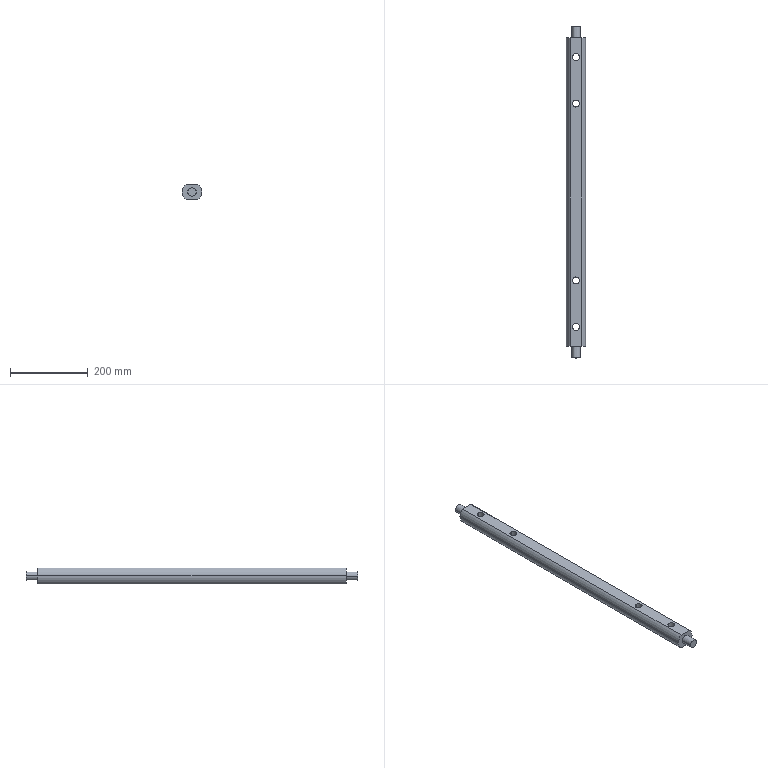Component | SolidWorks | FixedFrame-1 | 1 solid | 21 faces | box 50 x 856 x 40 mm | volume 1382352 mm3 | cylinder 15 | plane 6 | commonest cylinder face diameters 18 x8 22 x4 50 x3
build123d program:
from build123d import *

# Parameters (mm, degrees)
SKETCH1_R           = 25
BOSS_EXTRUDE1_DEPTH = 398
SKETCH2_R           = 11
BOSS_EXTRUDE2_DEPTH = 30
SKETCH3_W           = 60
SKETCH3_H           = 14.79
CUT_EXTRUDE1_DEPTH  = 827.756
SKETCH4_R           = 9
CUT_EXTRUDE2_DEPTH  = 656


with BuildPart() as part:
    # Sketch1 → Boss-Extrude1 (new, symmetric)
    with BuildSketch(Plane.XY):
        Circle(SKETCH1_R)
    extrude(amount=BOSS_EXTRUDE1_DEPTH, both=True)

    # Sketch2 → Boss-Extrude2 (add)
    with BuildSketch(Plane.XY.offset(398)):
        Circle(SKETCH2_R)
    extrude(amount=BOSS_EXTRUDE2_DEPTH)

    # Mirror1: part across plane


with BuildPart() as part_1:
    add(part.part)
    add(part.part.mirror(Plane.XY))

    # Sketch3 → Cut-Extrude1 (cut, through all)
    with BuildSketch(Plane.XY.offset(398)):
        with Locations((0, 27.395)):
            Rectangle(SKETCH3_W, SKETCH3_H)
        with Locations((0, -27.395)):
            Rectangle(SKETCH3_W, SKETCH3_H)
    extrude(amount=-CUT_EXTRUDE1_DEPTH, mode=Mode.SUBTRACT)

    # Sketch4 → Cut-Extrude2 (cut)
    with BuildSketch(Plane(origin=(0, 20, 0), x_dir=(1, 0, 0), z_dir=(0, 1, 0))):
        with Locations(Location((0, -228, 0), (0, 0, 270))):
            Circle(SKETCH4_R)
        with Locations(Location((0, -348, 0), (0, 0, 270))):
            Circle(SKETCH4_R)
        with Locations(Location((0, 348, 0), (0, 0, 270))):
            Circle(SKETCH4_R)
        with Locations(Location((0, 228, 0), (0, 0, 270))):
            Circle(SKETCH4_R)
    extrude(amount=-CUT_EXTRUDE2_DEPTH, mode=Mode.SUBTRACT)


solid = part_1.part

# Placed as in the assembly
solid = solid.moved(Location((-917, 0, -160), (90, 0, 0)))
STEP:
#1=COLOUR_RGB('',0.7922,0.8196,0.9333);
#2=FILL_AREA_STYLE_COLOUR('',#1);
#3=FILL_AREA_STYLE('',(#2));
#4=SURFACE_STYLE_FILL_AREA(#3);
#5=SURFACE_SIDE_STYLE('',(#4));
#6=SURFACE_STYLE_USAGE(.BOTH.,#5);
#7=PRESENTATION_STYLE_ASSIGNMENT((#6));
#8=CARTESIAN_POINT('',(-36.102,9.331,-7.087));
#9=VERTEX_POINT('',#8);
#10=CARTESIAN_POINT('',(-36.102,8.622,-7.087));
#11=VERTEX_POINT('',#10);
#12=CARTESIAN_POINT('',(-36.102,8.976,-7.087));
#13=DIRECTION('',(0.,-0.,1.));
#14=DIRECTION('',(0.,-1.,0.));
#15=AXIS2_PLACEMENT_3D('',#12,#13,#14);
#16=CIRCLE('',#15,0.3543);
#17=EDGE_CURVE('',#9,#11,#16,.T.);
#18=ORIENTED_EDGE('',*,*,#17,.F.);
#19=CARTESIAN_POINT('',(-36.102,9.331,-5.512));
#20=VERTEX_POINT('',#19);
#21=CARTESIAN_POINT('',(-36.102,9.331,-31.339));
#22=DIRECTION('',(0.,-0.,1.));
#23=VECTOR('',#22,39.37);
#24=LINE('',#21,#23);
#25=EDGE_CURVE('',#9,#20,#24,.T.);
#26=ORIENTED_EDGE('',*,*,#25,.T.);
#27=CARTESIAN_POINT('',(-36.102,8.622,-5.512));
#28=VERTEX_POINT('',#27);
#29=CARTESIAN_POINT('',(-36.102,8.976,-5.512));
#30=DIRECTION('',(0.,-0.,1.));
#31=DIRECTION('',(0.,1.,0.));
#32=AXIS2_PLACEMENT_3D('',#29,#30,#31);
#33=CIRCLE('',#32,0.3543);
#34=EDGE_CURVE('',#20,#28,#33,.T.);
#35=ORIENTED_EDGE('',*,*,#34,.T.);
#36=CARTESIAN_POINT('',(-36.102,8.622,-31.339));
#37=DIRECTION('',(0.,-0.,1.));
#38=VECTOR('',#37,39.37);
#39=LINE('',#36,#38);
#40=EDGE_CURVE('',#11,#28,#39,.T.);
#41=ORIENTED_EDGE('',*,*,#40,.F.);
#42=EDGE_LOOP('',(#18,#26,#35,#41));
#43=FACE_OUTER_BOUND('',#42,.T.);
#44=CARTESIAN_POINT('',(-36.102,8.976,-31.339));
#45=DIRECTION('',(0.,-0.,1.));
#46=DIRECTION('',(0.,-1.,0.));
#47=AXIS2_PLACEMENT_3D('',#44,#45,#46);
#48=CYLINDRICAL_SURFACE('',#47,0.3543);
#49=ADVANCED_FACE('',(#43),#48,.F.);
#50=CARTESIAN_POINT('',(-36.102,14.055,-7.087));
#51=VERTEX_POINT('',#50);
#52=CARTESIAN_POINT('',(-36.102,13.346,-7.087));
#53=VERTEX_POINT('',#52);
#54=CARTESIAN_POINT('',(-36.102,13.701,-7.087));
#55=DIRECTION('',(0.,-0.,1.));
#56=DIRECTION('',(0.,-1.,0.));
#57=AXIS2_PLACEMENT_3D('',#54,#55,#56);
#58=CIRCLE('',#57,0.3543);
#59=EDGE_CURVE('',#51,#53,#58,.T.);
#60=ORIENTED_EDGE('',*,*,#59,.F.);
#61=CARTESIAN_POINT('',(-36.102,14.055,-5.512));
#62=VERTEX_POINT('',#61);
#63=CARTESIAN_POINT('',(-36.102,14.055,-31.339));
#64=DIRECTION('',(0.,-0.,1.));
#65=VECTOR('',#64,39.37);
#66=LINE('',#63,#65);
#67=EDGE_CURVE('',#51,#62,#66,.T.);
#68=ORIENTED_EDGE('',*,*,#67,.T.);
#69=CARTESIAN_POINT('',(-36.102,13.346,-5.512));
#70=VERTEX_POINT('',#69);
#71=CARTESIAN_POINT('',(-36.102,13.701,-5.512));
#72=DIRECTION('',(0.,-0.,1.));
#73=DIRECTION('',(0.,1.,0.));
#74=AXIS2_PLACEMENT_3D('',#71,#72,#73);
#75=CIRCLE('',#74,0.3543);
#76=EDGE_CURVE('',#62,#70,#75,.T.);
#77=ORIENTED_EDGE('',*,*,#76,.T.);
#78=CARTESIAN_POINT('',(-36.102,13.346,-31.339));
#79=DIRECTION('',(0.,-0.,1.));
#80=VECTOR('',#79,39.37);
#81=LINE('',#78,#80);
#82=EDGE_CURVE('',#53,#70,#81,.T.);
#83=ORIENTED_EDGE('',*,*,#82,.F.);
#84=EDGE_LOOP('',(#60,#68,#77,#83));
#85=FACE_OUTER_BOUND('',#84,.T.);
#86=CARTESIAN_POINT('',(-36.102,13.701,-31.339));
#87=DIRECTION('',(0.,-0.,1.));
#88=DIRECTION('',(0.,-1.,0.));
#89=AXIS2_PLACEMENT_3D('',#86,#87,#88);
#90=CYLINDRICAL_SURFACE('',#89,0.3543);
#91=ADVANCED_FACE('',(#85),#90,.F.);
#92=CARTESIAN_POINT('',(-36.102,-13.346,-7.087));
#93=VERTEX_POINT('',#92);
#94=CARTESIAN_POINT('',(-36.102,-14.055,-7.087));
#95=VERTEX_POINT('',#94);
#96=CARTESIAN_POINT('',(-36.102,-13.701,-7.087));
#97=DIRECTION('',(0.,-0.,1.));
#98=DIRECTION('',(0.,-1.,0.));
#99=AXIS2_PLACEMENT_3D('',#96,#97,#98);
#100=CIRCLE('',#99,0.3543);
#101=EDGE_CURVE('',#93,#95,#100,.T.);
#102=ORIENTED_EDGE('',*,*,#101,.F.);
#103=CARTESIAN_POINT('',(-36.102,-13.346,-5.512));
#104=VERTEX_POINT('',#103);
#105=CARTESIAN_POINT('',(-36.102,-13.346,-31.339));
#106=DIRECTION('',(0.,-0.,1.));
#107=VECTOR('',#106,39.37);
#108=LINE('',#105,#107);
#109=EDGE_CURVE('',#93,#104,#108,.T.);
#110=ORIENTED_EDGE('',*,*,#109,.T.);
#111=CARTESIAN_POINT('',(-36.102,-14.055,-5.512));
#112=VERTEX_POINT('',#111);
#113=CARTESIAN_POINT('',(-36.102,-13.701,-5.512));
#114=DIRECTION('',(0.,-0.,1.));
#115=DIRECTION('',(0.,-1.,0.));
#116=AXIS2_PLACEMENT_3D('',#113,#114,#115);
#117=CIRCLE('',#116,0.3543);
#118=EDGE_CURVE('',#104,#112,#117,.T.);
#119=ORIENTED_EDGE('',*,*,#118,.T.);
#120=CARTESIAN_POINT('',(-36.102,-14.055,-31.339));
#121=DIRECTION('',(0.,-0.,1.));
#122=VECTOR('',#121,39.37);
#123=LINE('',#120,#122);
#124=EDGE_CURVE('',#95,#112,#123,.T.);
#125=ORIENTED_EDGE('',*,*,#124,.F.);
#126=EDGE_LOOP('',(#102,#110,#119,#125));
#127=FACE_OUTER_BOUND('',#126,.T.);
#128=CARTESIAN_POINT('',(-36.102,-13.701,-31.339));
#129=DIRECTION('',(0.,-0.,1.));
#130=DIRECTION('',(0.,-1.,0.));
#131=AXIS2_PLACEMENT_3D('',#128,#129,#130);
#132=CYLINDRICAL_SURFACE('',#131,0.3543);
#133=ADVANCED_FACE('',(#127),#132,.F.);
#134=CARTESIAN_POINT('',(-36.102,-8.622,-7.087));
#135=VERTEX_POINT('',#134);
#136=CARTESIAN_POINT('',(-36.102,-9.331,-7.087));
#137=VERTEX_POINT('',#136);
#138=CARTESIAN_POINT('',(-36.102,-8.976,-7.087));
#139=DIRECTION('',(0.,-0.,1.));
#140=DIRECTION('',(0.,-1.,0.));
#141=AXIS2_PLACEMENT_3D('',#138,#139,#140);
#142=CIRCLE('',#141,0.3543);
#143=EDGE_CURVE('',#135,#137,#142,.T.);
#144=ORIENTED_EDGE('',*,*,#143,.F.);
#145=CARTESIAN_POINT('',(-36.102,-8.622,-5.512));
#146=VERTEX_POINT('',#145);
#147=CARTESIAN_POINT('',(-36.102,-8.622,-31.339));
#148=DIRECTION('',(0.,-0.,1.));
#149=VECTOR('',#148,39.37);
#150=LINE('',#147,#149);
#151=EDGE_CURVE('',#135,#146,#150,.T.);
#152=ORIENTED_EDGE('',*,*,#151,.T.);
#153=CARTESIAN_POINT('',(-36.102,-9.331,-5.512));
#154=VERTEX_POINT('',#153);
#155=CARTESIAN_POINT('',(-36.102,-8.976,-5.512));
#156=DIRECTION('',(0.,-0.,1.));
#157=DIRECTION('',(0.,-1.,0.));
#158=AXIS2_PLACEMENT_3D('',#155,#156,#157);
#159=CIRCLE('',#158,0.3543);
#160=EDGE_CURVE('',#146,#154,#159,.T.);
#161=ORIENTED_EDGE('',*,*,#160,.T.);
#162=CARTESIAN_POINT('',(-36.102,-9.331,-31.339));
#163=DIRECTION('',(0.,-0.,1.));
#164=VECTOR('',#163,39.37);
#165=LINE('',#162,#164);
#166=EDGE_CURVE('',#137,#154,#165,.T.);
#167=ORIENTED_EDGE('',*,*,#166,.F.);
#168=EDGE_LOOP('',(#144,#152,#161,#167));
#169=FACE_OUTER_BOUND('',#168,.T.);
#170=CARTESIAN_POINT('',(-36.102,-8.976,-31.339));
#171=DIRECTION('',(0.,-0.,1.));
#172=DIRECTION('',(0.,-1.,0.));
#173=AXIS2_PLACEMENT_3D('',#170,#171,#172);
#174=CYLINDRICAL_SURFACE('',#173,0.3543);
#175=ADVANCED_FACE('',(#169),#174,.F.);
#176=CARTESIAN_POINT('',(-36.535,16.85,-6.299));
#177=VERTEX_POINT('',#176);
#178=CARTESIAN_POINT('',(-35.669,16.85,-6.299));
#179=VERTEX_POINT('',#178);
#180=CARTESIAN_POINT('',(-36.102,16.85,-6.299));
#181=DIRECTION('',(-0.,-1.,-0.));
#182=DIRECTION('',(1.,0.,-0.));
#183=AXIS2_PLACEMENT_3D('',#180,#181,#182);
#184=CIRCLE('',#183,0.4331);
#185=EDGE_CURVE('',#177,#179,#184,.T.);
#186=ORIENTED_EDGE('',*,*,#185,.T.);
#187=CARTESIAN_POINT('',(-35.669,15.669,-6.299));
#188=VERTEX_POINT('',#187);
#189=CARTESIAN_POINT('',(-35.669,16.85,-6.299));
#190=DIRECTION('',(-0.,-1.,-0.));
#191=VECTOR('',#190,39.37);
#192=LINE('',#189,#191);
#193=EDGE_CURVE('',#179,#188,#192,.T.);
#194=ORIENTED_EDGE('',*,*,#193,.T.);
#195=CARTESIAN_POINT('',(-36.535,15.669,-6.299));
#196=VERTEX_POINT('',#195);
#197=CARTESIAN_POINT('',(-36.102,15.669,-6.299));
#198=DIRECTION('',(0.,1.,0.));
#199=DIRECTION('',(1.,0.,-0.));
#200=AXIS2_PLACEMENT_3D('',#197,#198,#199);
#201=CIRCLE('',#200,0.4331);
#202=EDGE_CURVE('',#188,#196,#201,.T.);
#203=ORIENTED_EDGE('',*,*,#202,.T.);
#204=CARTESIAN_POINT('',(-36.535,16.85,-6.299));
#205=DIRECTION('',(-0.,-1.,-0.));
#206=VECTOR('',#205,39.37);
#207=LINE('',#204,#206);
#208=EDGE_CURVE('',#177,#196,#207,.T.);
#209=ORIENTED_EDGE('',*,*,#208,.F.);
#210=EDGE_LOOP('',(#186,#194,#203,#209));
#211=FACE_OUTER_BOUND('',#210,.T.);
#212=CARTESIAN_POINT('',(-36.102,16.85,-6.299));
#213=DIRECTION('',(-0.,-1.,-0.));
#214=DIRECTION('',(-1.,0.,0.));
#215=AXIS2_PLACEMENT_3D('',#212,#213,#214);
#216=CYLINDRICAL_SURFACE('',#215,0.4331);
#217=ADVANCED_FACE('',(#211),#216,.T.);
#218=CARTESIAN_POINT('',(-35.669,-16.85,-6.299));
#219=VERTEX_POINT('',#218);
#220=CARTESIAN_POINT('',(-36.535,-16.85,-6.299));
#221=VERTEX_POINT('',#220);
#222=CARTESIAN_POINT('',(-36.102,-16.85,-6.299));
#223=DIRECTION('',(-0.,-1.,-0.));
#224=DIRECTION('',(1.,0.,-0.));
#225=AXIS2_PLACEMENT_3D('',#222,#223,#224);
#226=CIRCLE('',#225,0.4331);
#227=EDGE_CURVE('',#219,#221,#226,.T.);
#228=ORIENTED_EDGE('',*,*,#227,.F.);
#229=CARTESIAN_POINT('',(-35.669,-15.669,-6.299));
#230=VERTEX_POINT('',#229);
#231=CARTESIAN_POINT('',(-35.669,-16.85,-6.299));
#232=DIRECTION('',(0.,1.,0.));
#233=VECTOR('',#232,39.37);
#234=LINE('',#231,#233);
#235=EDGE_CURVE('',#219,#230,#234,.T.);
#236=ORIENTED_EDGE('',*,*,#235,.T.);
#237=CARTESIAN_POINT('',(-36.535,-15.669,-6.299));
#238=VERTEX_POINT('',#237);
#239=CARTESIAN_POINT('',(-36.102,-15.669,-6.299));
#240=DIRECTION('',(-0.,-1.,-0.));
#241=DIRECTION('',(1.,0.,-0.));
#242=AXIS2_PLACEMENT_3D('',#239,#240,#241);
#243=CIRCLE('',#242,0.4331);
#244=EDGE_CURVE('',#230,#238,#243,.T.);
#245=ORIENTED_EDGE('',*,*,#244,.T.);
#246=CARTESIAN_POINT('',(-36.535,-16.85,-6.299));
#247=DIRECTION('',(0.,1.,0.));
#248=VECTOR('',#247,39.37);
#249=LINE('',#246,#248);
#250=EDGE_CURVE('',#221,#238,#249,.T.);
#251=ORIENTED_EDGE('',*,*,#250,.F.);
#252=EDGE_LOOP('',(#228,#236,#245,#251));
#253=FACE_OUTER_BOUND('',#252,.T.);
#254=CARTESIAN_POINT('',(-36.102,-16.85,-6.299));
#255=DIRECTION('',(0.,1.,0.));
#256=DIRECTION('',(-1.,0.,0.));
#257=AXIS2_PLACEMENT_3D('',#254,#255,#256);
#258=CYLINDRICAL_SURFACE('',#257,0.4331);
#259=ADVANCED_FACE('',(#253),#258,.T.);
#260=CARTESIAN_POINT('',(-37.087,-15.669,-6.299));
#261=VERTEX_POINT('',#260);
#262=CARTESIAN_POINT('',(-36.693,-15.669,-7.087));
#263=VERTEX_POINT('',#262);
#264=CARTESIAN_POINT('',(-36.102,-15.669,-6.299));
#265=DIRECTION('',(-0.,-1.,-0.));
#266=DIRECTION('',(1.,0.,-0.));
#267=AXIS2_PLACEMENT_3D('',#264,#265,#266);
#268=CIRCLE('',#267,0.9843);
#269=EDGE_CURVE('',#261,#263,#268,.T.);
#270=ORIENTED_EDGE('',*,*,#269,.F.);
#271=CARTESIAN_POINT('',(-37.087,15.669,-6.299));
#272=VERTEX_POINT('',#271);
#273=CARTESIAN_POINT('',(-37.087,-15.669,-6.299));
#274=DIRECTION('',(0.,1.,0.));
#275=VECTOR('',#274,39.37);
#276=LINE('',#273,#275);
#277=EDGE_CURVE('',#261,#272,#276,.T.);
#278=ORIENTED_EDGE('',*,*,#277,.T.);
#279=CARTESIAN_POINT('',(-36.693,15.669,-7.087));
#280=VERTEX_POINT('',#279);
#281=CARTESIAN_POINT('',(-36.102,15.669,-6.299));
#282=DIRECTION('',(-0.,-1.,-0.));
#283=DIRECTION('',(1.,0.,-0.));
#284=AXIS2_PLACEMENT_3D('',#281,#282,#283);
#285=CIRCLE('',#284,0.9843);
#286=EDGE_CURVE('',#272,#280,#285,.T.);
#287=ORIENTED_EDGE('',*,*,#286,.T.);
#288=CARTESIAN_POINT('',(-36.693,-15.669,-7.087));
#289=DIRECTION('',(-0.,-1.,-0.));
#290=VECTOR('',#289,39.37);
#291=LINE('',#288,#290);
#292=EDGE_CURVE('',#280,#263,#291,.T.);
#293=ORIENTED_EDGE('',*,*,#292,.T.);
#294=EDGE_LOOP('',(#270,#278,#287,#293));
#295=FACE_OUTER_BOUND('',#294,.T.);
#296=CARTESIAN_POINT('',(-36.102,-15.669,-6.299));
#297=DIRECTION('',(0.,1.,0.));
#298=DIRECTION('',(-1.,0.,0.));
#299=AXIS2_PLACEMENT_3D('',#296,#297,#298);
#300=CYLINDRICAL_SURFACE('',#299,0.9843);
#301=ADVANCED_FACE('',(#295),#300,.T.);
#302=CARTESIAN_POINT('',(-35.512,-15.669,-7.087));
#303=VERTEX_POINT('',#302);
#304=CARTESIAN_POINT('',(-35.512,-15.669,-5.512));
#305=VERTEX_POINT('',#304);
#306=CARTESIAN_POINT('',(-36.102,-15.669,-6.299));
#307=DIRECTION('',(-0.,-1.,-0.));
#308=DIRECTION('',(1.,0.,-0.));
#309=AXIS2_PLACEMENT_3D('',#306,#307,#308);
#310=CIRCLE('',#309,0.9843);
#311=EDGE_CURVE('',#303,#305,#310,.T.);
#312=ORIENTED_EDGE('',*,*,#311,.F.);
#313=CARTESIAN_POINT('',(-35.512,15.669,-7.087));
#314=VERTEX_POINT('',#313);
#315=CARTESIAN_POINT('',(-35.512,-15.669,-7.087));
#316=DIRECTION('',(0.,1.,0.));
#317=VECTOR('',#316,39.37);
#318=LINE('',#315,#317);
#319=EDGE_CURVE('',#303,#314,#318,.T.);
#320=ORIENTED_EDGE('',*,*,#319,.T.);
#321=CARTESIAN_POINT('',(-35.512,15.669,-5.512));
#322=VERTEX_POINT('',#321);
#323=CARTESIAN_POINT('',(-36.102,15.669,-6.299));
#324=DIRECTION('',(-0.,-1.,-0.));
#325=DIRECTION('',(1.,0.,-0.));
#326=AXIS2_PLACEMENT_3D('',#323,#324,#325);
#327=CIRCLE('',#326,0.9843);
#328=EDGE_CURVE('',#314,#322,#327,.T.);
#329=ORIENTED_EDGE('',*,*,#328,.T.);
#330=CARTESIAN_POINT('',(-35.512,-15.669,-5.512));
#331=DIRECTION('',(-0.,-1.,-0.));
#332=VECTOR('',#331,39.37);
#333=LINE('',#330,#332);
#334=EDGE_CURVE('',#322,#305,#333,.T.);
#335=ORIENTED_EDGE('',*,*,#334,.T.);
#336=EDGE_LOOP('',(#312,#320,#329,#335));
#337=FACE_OUTER_BOUND('',#336,.T.);
#338=CARTESIAN_POINT('',(-36.102,-15.669,-6.299));
#339=DIRECTION('',(0.,1.,0.));
#340=DIRECTION('',(-1.,0.,0.));
#341=AXIS2_PLACEMENT_3D('',#338,#339,#340);
#342=CYLINDRICAL_SURFACE('',#341,0.9843);
#343=ADVANCED_FACE('',(#337),#342,.T.);
#344=ORIENTED_EDGE('',*,*,#328,.F.);
#345=CARTESIAN_POINT('',(-36.102,15.669,-7.087));
#346=DIRECTION('',(-1.,0.,0.));
#347=VECTOR('',#346,39.37);
#348=LINE('',#345,#347);
#349=EDGE_CURVE('',#314,#280,#348,.T.);
#350=ORIENTED_EDGE('',*,*,#349,.T.);
#351=ORIENTED_EDGE('',*,*,#286,.F.);
#352=CARTESIAN_POINT('',(-36.693,15.669,-5.512));
#353=VERTEX_POINT('',#352);
#354=CARTESIAN_POINT('',(-36.102,15.669,-6.299));
#355=DIRECTION('',(-0.,-1.,-0.));
#356=DIRECTION('',(1.,0.,-0.));
#357=AXIS2_PLACEMENT_3D('',#354,#355,#356);
#358=CIRCLE('',#357,0.9843);
#359=EDGE_CURVE('',#353,#272,#358,.T.);
#360=ORIENTED_EDGE('',*,*,#359,.F.);
#361=CARTESIAN_POINT('',(-36.102,15.669,-5.512));
#362=DIRECTION('',(1.,-0.,-0.));
#363=VECTOR('',#362,39.37);
#364=LINE('',#361,#363);
#365=EDGE_CURVE('',#353,#322,#364,.T.);
#366=ORIENTED_EDGE('',*,*,#365,.T.);
#367=EDGE_LOOP('',(#344,#350,#351,#360,#366));
#368=FACE_OUTER_BOUND('',#367,.T.);
#369=CARTESIAN_POINT('',(-36.102,15.669,-6.299));
#370=DIRECTION('',(0.,1.,0.));
#371=DIRECTION('',(1.,0.,-0.));
#372=AXIS2_PLACEMENT_3D('',#369,#370,#371);
#373=CIRCLE('',#372,0.4331);
#374=EDGE_CURVE('',#196,#188,#373,.T.);
#375=ORIENTED_EDGE('',*,*,#374,.F.);
#376=ORIENTED_EDGE('',*,*,#202,.F.);
#377=EDGE_LOOP('',(#375,#376));
#378=FACE_BOUND('',#377,.T.);
#379=CARTESIAN_POINT('',(-36.102,15.669,-6.299));
#380=DIRECTION('',(-0.,-1.,-0.));
#381=DIRECTION('',(1.,-0.,-0.));
#382=AXIS2_PLACEMENT_3D('',#379,#380,#381);
#383=PLANE('',#382);
#384=ADVANCED_FACE('',(#368,#378),#383,.F.);
#385=CARTESIAN_POINT('',(-37.283,-15.669,-7.087));
#386=DIRECTION('',(-1.,0.,0.));
#387=VECTOR('',#386,39.37);
#388=LINE('',#385,#387);
#389=EDGE_CURVE('',#303,#263,#388,.T.);
#390=ORIENTED_EDGE('',*,*,#389,.F.);
#391=ORIENTED_EDGE('',*,*,#311,.T.);
#392=CARTESIAN_POINT('',(-36.693,-15.669,-5.512));
#393=VERTEX_POINT('',#392);
#394=CARTESIAN_POINT('',(-37.283,-15.669,-5.512));
#395=DIRECTION('',(1.,-0.,-0.));
#396=VECTOR('',#395,39.37);
#397=LINE('',#394,#396);
#398=EDGE_CURVE('',#393,#305,#397,.T.);
#399=ORIENTED_EDGE('',*,*,#398,.F.);
#400=CARTESIAN_POINT('',(-36.102,-15.669,-6.299));
#401=DIRECTION('',(-0.,-1.,-0.));
#402=DIRECTION('',(1.,0.,-0.));
#403=AXIS2_PLACEMENT_3D('',#400,#401,#402);
#404=CIRCLE('',#403,0.9843);
#405=EDGE_CURVE('',#393,#261,#404,.T.);
#406=ORIENTED_EDGE('',*,*,#405,.T.);
#407=ORIENTED_EDGE('',*,*,#269,.T.);
#408=EDGE_LOOP('',(#390,#391,#399,#406,#407));
#409=FACE_OUTER_BOUND('',#408,.T.);
#410=CARTESIAN_POINT('',(-36.102,-15.669,-6.299));
#411=DIRECTION('',(-0.,-1.,-0.));
#412=DIRECTION('',(1.,0.,-0.));
#413=AXIS2_PLACEMENT_3D('',#410,#411,#412);
#414=CIRCLE('',#413,0.4331);
#415=EDGE_CURVE('',#238,#230,#414,.T.);
#416=ORIENTED_EDGE('',*,*,#415,.F.);
#417=ORIENTED_EDGE('',*,*,#244,.F.);
#418=EDGE_LOOP('',(#416,#417));
#419=FACE_BOUND('',#418,.T.);
#420=CARTESIAN_POINT('',(-36.102,-15.669,-6.299));
#421=DIRECTION('',(-0.,-1.,-0.));
#422=DIRECTION('',(1.,-0.,-0.));
#423=AXIS2_PLACEMENT_3D('',#420,#421,#422);
#424=PLANE('',#423);
#425=ADVANCED_FACE('',(#409,#419),#424,.T.);
#426=ORIENTED_EDGE('',*,*,#277,.F.);
#427=ORIENTED_EDGE('',*,*,#405,.F.);
#428=CARTESIAN_POINT('',(-36.693,-15.669,-5.512));
#429=DIRECTION('',(0.,1.,0.));
#430=VECTOR('',#429,39.37);
#431=LINE('',#428,#430);
#432=EDGE_CURVE('',#393,#353,#431,.T.);
#433=ORIENTED_EDGE('',*,*,#432,.T.);
#434=ORIENTED_EDGE('',*,*,#359,.T.);
#435=EDGE_LOOP('',(#426,#427,#433,#434));
#436=FACE_OUTER_BOUND('',#435,.T.);
#437=CARTESIAN_POINT('',(-36.102,-15.669,-6.299));
#438=DIRECTION('',(0.,1.,0.));
#439=DIRECTION('',(-1.,0.,0.));
#440=AXIS2_PLACEMENT_3D('',#437,#438,#439);
#441=CYLINDRICAL_SURFACE('',#440,0.9843);
#442=ADVANCED_FACE('',(#436),#441,.T.);
#443=ORIENTED_EDGE('',*,*,#235,.F.);
#444=CARTESIAN_POINT('',(-36.102,-16.85,-6.299));
#445=DIRECTION('',(-0.,-1.,-0.));
#446=DIRECTION('',(1.,0.,-0.));
#447=AXIS2_PLACEMENT_3D('',#444,#445,#446);
#448=CIRCLE('',#447,0.4331);
#449=EDGE_CURVE('',#221,#219,#448,.T.);
#450=ORIENTED_EDGE('',*,*,#449,.F.);
#451=ORIENTED_EDGE('',*,*,#250,.T.);
#452=ORIENTED_EDGE('',*,*,#415,.T.);
#453=EDGE_LOOP('',(#443,#450,#451,#452));
#454=FACE_OUTER_BOUND('',#453,.T.);
#455=CARTESIAN_POINT('',(-36.102,-16.85,-6.299));
#456=DIRECTION('',(0.,1.,0.));
#457=DIRECTION('',(-1.,0.,0.));
#458=AXIS2_PLACEMENT_3D('',#455,#456,#457);
#459=CYLINDRICAL_SURFACE('',#458,0.4331);
#460=ADVANCED_FACE('',(#454),#459,.T.);
#461=ORIENTED_EDGE('',*,*,#449,.T.);
#462=ORIENTED_EDGE('',*,*,#227,.T.);
#463=EDGE_LOOP('',(#461,#462));
#464=FACE_OUTER_BOUND('',#463,.T.);
#465=CARTESIAN_POINT('',(-36.102,-16.85,-6.299));
#466=DIRECTION('',(-0.,-1.,-0.));
#467=DIRECTION('',(1.,-0.,-0.));
#468=AXIS2_PLACEMENT_3D('',#465,#466,#467);
#469=PLANE('',#468);
#470=ADVANCED_FACE('',(#464),#469,.T.);
#471=ORIENTED_EDGE('',*,*,#193,.F.);
#472=CARTESIAN_POINT('',(-36.102,16.85,-6.299));
#473=DIRECTION('',(-0.,-1.,-0.));
#474=DIRECTION('',(1.,0.,-0.));
#475=AXIS2_PLACEMENT_3D('',#472,#473,#474);
#476=CIRCLE('',#475,0.4331);
#477=EDGE_CURVE('',#179,#177,#476,.T.);
#478=ORIENTED_EDGE('',*,*,#477,.T.);
#479=ORIENTED_EDGE('',*,*,#208,.T.);
#480=ORIENTED_EDGE('',*,*,#374,.T.);
#481=EDGE_LOOP('',(#471,#478,#479,#480));
#482=FACE_OUTER_BOUND('',#481,.T.);
#483=CARTESIAN_POINT('',(-36.102,16.85,-6.299));
#484=DIRECTION('',(-0.,-1.,-0.));
#485=DIRECTION('',(-1.,0.,0.));
#486=AXIS2_PLACEMENT_3D('',#483,#484,#485);
#487=CYLINDRICAL_SURFACE('',#486,0.4331);
#488=ADVANCED_FACE('',(#482),#487,.T.);
#489=ORIENTED_EDGE('',*,*,#185,.F.);
#490=ORIENTED_EDGE('',*,*,#477,.F.);
#491=EDGE_LOOP('',(#489,#490));
#492=FACE_OUTER_BOUND('',#491,.T.);
#493=CARTESIAN_POINT('',(-36.102,16.85,-6.299));
#494=DIRECTION('',(0.,1.,0.));
#495=DIRECTION('',(1.,-0.,-0.));
#496=AXIS2_PLACEMENT_3D('',#493,#494,#495);
#497=PLANE('',#496);
#498=ADVANCED_FACE('',(#492),#497,.T.);
#499=CARTESIAN_POINT('',(-36.102,8.976,-5.512));
#500=DIRECTION('',(0.,-0.,1.));
#501=DIRECTION('',(0.,1.,0.));
#502=AXIS2_PLACEMENT_3D('',#499,#500,#501);
#503=CIRCLE('',#502,0.3543);
#504=EDGE_CURVE('',#28,#20,#503,.T.);
#505=ORIENTED_EDGE('',*,*,#504,.F.);
#506=ORIENTED_EDGE('',*,*,#34,.F.);
#507=EDGE_LOOP('',(#505,#506));
#508=FACE_BOUND('',#507,.T.);
#509=CARTESIAN_POINT('',(-36.102,13.701,-5.512));
#510=DIRECTION('',(0.,-0.,1.));
#511=DIRECTION('',(0.,1.,0.));
#512=AXIS2_PLACEMENT_3D('',#509,#510,#511);
#513=CIRCLE('',#512,0.3543);
#514=EDGE_CURVE('',#70,#62,#513,.T.);
#515=ORIENTED_EDGE('',*,*,#514,.F.);
#516=ORIENTED_EDGE('',*,*,#76,.F.);
#517=EDGE_LOOP('',(#515,#516));
#518=FACE_BOUND('',#517,.T.);
#519=CARTESIAN_POINT('',(-36.102,-13.701,-5.512));
#520=DIRECTION('',(0.,-0.,1.));
#521=DIRECTION('',(0.,-1.,0.));
#522=AXIS2_PLACEMENT_3D('',#519,#520,#521);
#523=CIRCLE('',#522,0.3543);
#524=EDGE_CURVE('',#112,#104,#523,.T.);
#525=ORIENTED_EDGE('',*,*,#524,.F.);
#526=ORIENTED_EDGE('',*,*,#118,.F.);
#527=EDGE_LOOP('',(#525,#526));
#528=FACE_BOUND('',#527,.T.);
#529=CARTESIAN_POINT('',(-36.102,-8.976,-5.512));
#530=DIRECTION('',(0.,-0.,1.));
#531=DIRECTION('',(0.,-1.,0.));
#532=AXIS2_PLACEMENT_3D('',#529,#530,#531);
#533=CIRCLE('',#532,0.3543);
#534=EDGE_CURVE('',#154,#146,#533,.T.);
#535=ORIENTED_EDGE('',*,*,#534,.F.);
#536=ORIENTED_EDGE('',*,*,#160,.F.);
#537=EDGE_LOOP('',(#535,#536));
#538=FACE_BOUND('',#537,.T.);
#539=ORIENTED_EDGE('',*,*,#398,.T.);
#540=ORIENTED_EDGE('',*,*,#334,.F.);
#541=ORIENTED_EDGE('',*,*,#365,.F.);
#542=ORIENTED_EDGE('',*,*,#432,.F.);
#543=EDGE_LOOP('',(#539,#540,#541,#542));
#544=FACE_OUTER_BOUND('',#543,.T.);
#545=CARTESIAN_POINT('',(-37.283,16.85,-5.512));
#546=DIRECTION('',(-0.,0.,-1.));
#547=DIRECTION('',(0.,1.,0.));
#548=AXIS2_PLACEMENT_3D('',#545,#546,#547);
#549=PLANE('',#548);
#550=ADVANCED_FACE('',(#508,#518,#528,#538,#544),#549,.F.);
#551=CARTESIAN_POINT('',(-36.102,8.976,-7.087));
#552=DIRECTION('',(0.,-0.,1.));
#553=DIRECTION('',(0.,-1.,0.));
#554=AXIS2_PLACEMENT_3D('',#551,#552,#553);
#555=CIRCLE('',#554,0.3543);
#556=EDGE_CURVE('',#11,#9,#555,.T.);
#557=ORIENTED_EDGE('',*,*,#556,.T.);
#558=ORIENTED_EDGE('',*,*,#17,.T.);
#559=EDGE_LOOP('',(#557,#558));
#560=FACE_BOUND('',#559,.T.);
#561=CARTESIAN_POINT('',(-36.102,13.701,-7.087));
#562=DIRECTION('',(0.,-0.,1.));
#563=DIRECTION('',(0.,-1.,0.));
#564=AXIS2_PLACEMENT_3D('',#561,#562,#563);
#565=CIRCLE('',#564,0.3543);
#566=EDGE_CURVE('',#53,#51,#565,.T.);
#567=ORIENTED_EDGE('',*,*,#566,.T.);
#568=ORIENTED_EDGE('',*,*,#59,.T.);
#569=EDGE_LOOP('',(#567,#568));
#570=FACE_BOUND('',#569,.T.);
#571=CARTESIAN_POINT('',(-36.102,-13.701,-7.087));
#572=DIRECTION('',(0.,-0.,1.));
#573=DIRECTION('',(0.,-1.,0.));
#574=AXIS2_PLACEMENT_3D('',#571,#572,#573);
#575=CIRCLE('',#574,0.3543);
#576=EDGE_CURVE('',#95,#93,#575,.T.);
#577=ORIENTED_EDGE('',*,*,#576,.T.);
#578=ORIENTED_EDGE('',*,*,#101,.T.);
#579=EDGE_LOOP('',(#577,#578));
#580=FACE_BOUND('',#579,.T.);
#581=CARTESIAN_POINT('',(-36.102,-8.976,-7.087));
#582=DIRECTION('',(0.,-0.,1.));
#583=DIRECTION('',(0.,-1.,0.));
#584=AXIS2_PLACEMENT_3D('',#581,#582,#583);
#585=CIRCLE('',#584,0.3543);
#586=EDGE_CURVE('',#137,#135,#585,.T.);
#587=ORIENTED_EDGE('',*,*,#586,.T.);
#588=ORIENTED_EDGE('',*,*,#143,.T.);
#589=EDGE_LOOP('',(#587,#588));
#590=FACE_BOUND('',#589,.T.);
#591=ORIENTED_EDGE('',*,*,#389,.T.);
#592=ORIENTED_EDGE('',*,*,#292,.F.);
#593=ORIENTED_EDGE('',*,*,#349,.F.);
#594=ORIENTED_EDGE('',*,*,#319,.F.);
#595=EDGE_LOOP('',(#591,#592,#593,#594));
#596=FACE_OUTER_BOUND('',#595,.T.);
#597=CARTESIAN_POINT('',(-37.283,16.85,-7.087));
#598=DIRECTION('',(0.,-0.,1.));
#599=DIRECTION('',(-0.,-1.,-0.));
#600=AXIS2_PLACEMENT_3D('',#597,#598,#599);
#601=PLANE('',#600);
#602=ADVANCED_FACE('',(#560,#570,#580,#590,#596),#601,.F.);
#603=ORIENTED_EDGE('',*,*,#151,.F.);
#604=ORIENTED_EDGE('',*,*,#586,.F.);
#605=ORIENTED_EDGE('',*,*,#166,.T.);
#606=ORIENTED_EDGE('',*,*,#534,.T.);
#607=EDGE_LOOP('',(#603,#604,#605,#606));
#608=FACE_OUTER_BOUND('',#607,.T.);
#609=CARTESIAN_POINT('',(-36.102,-8.976,-31.339));
#610=DIRECTION('',(0.,-0.,1.));
#611=DIRECTION('',(0.,-1.,0.));
#612=AXIS2_PLACEMENT_3D('',#609,#610,#611);
#613=CYLINDRICAL_SURFACE('',#612,0.3543);
#614=ADVANCED_FACE('',(#608),#613,.F.);
#615=ORIENTED_EDGE('',*,*,#109,.F.);
#616=ORIENTED_EDGE('',*,*,#576,.F.);
#617=ORIENTED_EDGE('',*,*,#124,.T.);
#618=ORIENTED_EDGE('',*,*,#524,.T.);
#619=EDGE_LOOP('',(#615,#616,#617,#618));
#620=FACE_OUTER_BOUND('',#619,.T.);
#621=CARTESIAN_POINT('',(-36.102,-13.701,-31.339));
#622=DIRECTION('',(0.,-0.,1.));
#623=DIRECTION('',(0.,-1.,0.));
#624=AXIS2_PLACEMENT_3D('',#621,#622,#623);
#625=CYLINDRICAL_SURFACE('',#624,0.3543);
#626=ADVANCED_FACE('',(#620),#625,.F.);
#627=ORIENTED_EDGE('',*,*,#67,.F.);
#628=ORIENTED_EDGE('',*,*,#566,.F.);
#629=ORIENTED_EDGE('',*,*,#82,.T.);
#630=ORIENTED_EDGE('',*,*,#514,.T.);
#631=EDGE_LOOP('',(#627,#628,#629,#630));
#632=FACE_OUTER_BOUND('',#631,.T.);
#633=CARTESIAN_POINT('',(-36.102,13.701,-31.339));
#634=DIRECTION('',(0.,-0.,1.));
#635=DIRECTION('',(0.,-1.,0.));
#636=AXIS2_PLACEMENT_3D('',#633,#634,#635);
#637=CYLINDRICAL_SURFACE('',#636,0.3543);
#638=ADVANCED_FACE('',(#632),#637,.F.);
#639=ORIENTED_EDGE('',*,*,#25,.F.);
#640=ORIENTED_EDGE('',*,*,#556,.F.);
#641=ORIENTED_EDGE('',*,*,#40,.T.);
#642=ORIENTED_EDGE('',*,*,#504,.T.);
#643=EDGE_LOOP('',(#639,#640,#641,#642));
#644=FACE_OUTER_BOUND('',#643,.T.);
#645=CARTESIAN_POINT('',(-36.102,8.976,-31.339));
#646=DIRECTION('',(0.,-0.,1.));
#647=DIRECTION('',(0.,-1.,0.));
#648=AXIS2_PLACEMENT_3D('',#645,#646,#647);
#649=CYLINDRICAL_SURFACE('',#648,0.3543);
#650=ADVANCED_FACE('',(#644),#649,.F.);
#651=CLOSED_SHELL('',(#49,#91,#133,#175,#217,#259,#301,#343,#384,#425,#442,#460,#470,#488,#498,#550,#602,#614,#626,#638,#650));
#652=MANIFOLD_SOLID_BREP('',#651);
#653=STYLED_ITEM('',(#7),#652);
#654=(LENGTH_UNIT()NAMED_UNIT(*)SI_UNIT($,.METRE.));
#655=LENGTH_MEASURE_WITH_UNIT(LENGTH_MEASURE(0.0254),#654);
#656=DIMENSIONAL_EXPONENTS(1.,0.,0.,0.,0.,0.,0.);
#657=(CONVERSION_BASED_UNIT('',#655)LENGTH_UNIT()NAMED_UNIT(#656));
#658=UNCERTAINTY_MEASURE_WITH_UNIT(LENGTH_MEASURE(0.00001),#657,'','');
#659=(NAMED_UNIT(*)PLANE_ANGLE_UNIT()SI_UNIT($,.RADIAN.));
#660=(NAMED_UNIT(*)SI_UNIT($,.STERADIAN.)SOLID_ANGLE_UNIT());
#661=(GEOMETRIC_REPRESENTATION_CONTEXT(3)GLOBAL_UNCERTAINTY_ASSIGNED_CONTEXT((#658))GLOBAL_UNIT_ASSIGNED_CONTEXT((#657,#659,#660))REPRESENTATION_CONTEXT('',''));
#662=MECHANICAL_DESIGN_GEOMETRIC_PRESENTATION_REPRESENTATION('',(#653),#661);
#663=PRESENTATION_LAYER_ASSIGNMENT('','',(#653));
#664=CARTESIAN_POINT('',(0.,0.,0.));
#665=DIRECTION('',(0.,0.,1.));
#666=DIRECTION('',(1.,0.,0.));
#667=AXIS2_PLACEMENT_3D('',#664,#665,#666);
#668=(LENGTH_UNIT()NAMED_UNIT(*)SI_UNIT($,.METRE.));
#669=LENGTH_MEASURE_WITH_UNIT(LENGTH_MEASURE(0.0254),#668);
#670=DIMENSIONAL_EXPONENTS(1.,0.,0.,0.,0.,0.,0.);
#671=(CONVERSION_BASED_UNIT('',#669)LENGTH_UNIT()NAMED_UNIT(#670));
#672=UNCERTAINTY_MEASURE_WITH_UNIT(LENGTH_MEASURE(0.00001),#671,'','');
#673=(NAMED_UNIT(*)PLANE_ANGLE_UNIT()SI_UNIT($,.RADIAN.));
#674=(NAMED_UNIT(*)SI_UNIT($,.STERADIAN.)SOLID_ANGLE_UNIT());
#675=(GEOMETRIC_REPRESENTATION_CONTEXT(3)GLOBAL_UNCERTAINTY_ASSIGNED_CONTEXT((#672))GLOBAL_UNIT_ASSIGNED_CONTEXT((#671,#673,#674))REPRESENTATION_CONTEXT('',''));
#676=ADVANCED_BREP_SHAPE_REPRESENTATION('',(#652,#667),#675);